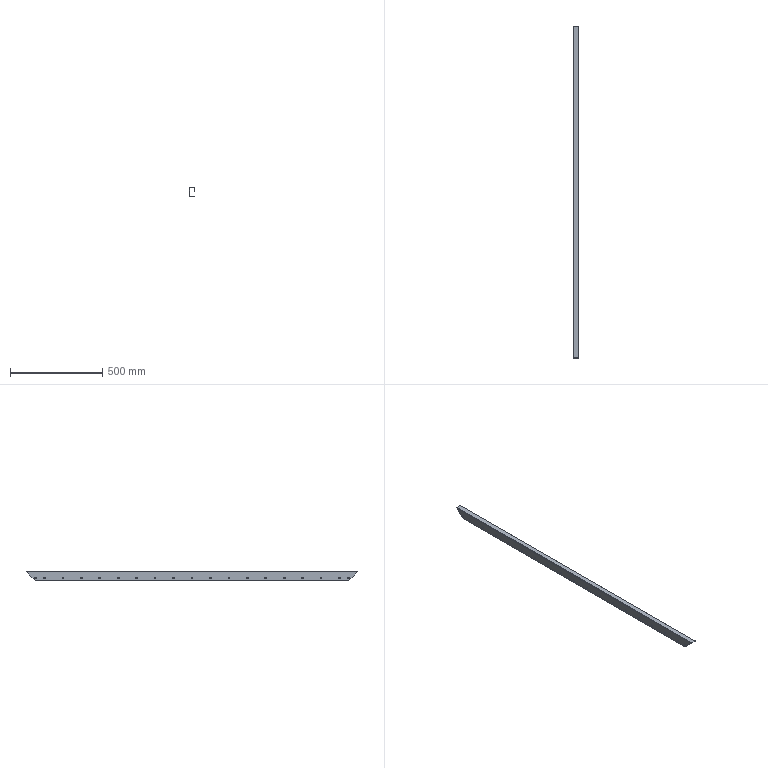Component | SolidWorks | KSHE-016.1.SLDPRT-1_KSHE-016.001-1 | 1 solid | 260 faces | volume 434069 mm3 | cylinder 226 | plane 30 | spline 4 | commonest cylinder face diameters 9 x208 5.1 x12 4.2 x3 0.2 x3